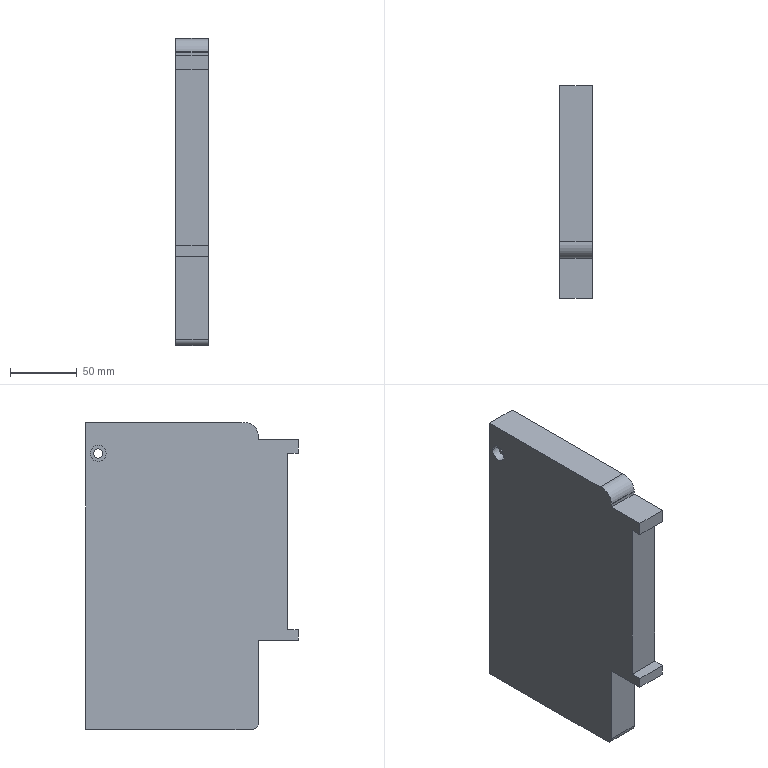Component | SolidWorks | 11-2 | 1 solid | 36 faces | box 24 x 159.37 x 230.25 mm | volume 437688 mm3 | plane 25 | cylinder 11 | commonest cylinder face diameters 20 x3 12 x2 7 x2 24 x2 4 x1 9.34 x1
STEP:
#1=COLOUR_RGB('',0.7922,0.8196,0.9333);
#2=FILL_AREA_STYLE_COLOUR('',#1);
#3=FILL_AREA_STYLE('',(#2));
#4=SURFACE_STYLE_FILL_AREA(#3);
#5=SURFACE_SIDE_STYLE('',(#4));
#6=SURFACE_STYLE_USAGE(.BOTH.,#5);
#7=PRESENTATION_STYLE_ASSIGNMENT((#6));
#8=CARTESIAN_POINT('',(-7.758,16.141,29.439));
#9=VERTEX_POINT('',#8);
#10=CARTESIAN_POINT('',(-7.758,16.614,29.439));
#11=VERTEX_POINT('',#10);
#12=CARTESIAN_POINT('',(-7.758,16.378,29.439));
#13=DIRECTION('',(1.,0.,-0.));
#14=DIRECTION('',(0.,-1.,0.));
#15=AXIS2_PLACEMENT_3D('',#12,#13,#14);
#16=CIRCLE('',#15,0.2362);
#17=EDGE_CURVE('',#9,#11,#16,.T.);
#18=ORIENTED_EDGE('',*,*,#17,.T.);
#19=CARTESIAN_POINT('',(-7.994,16.614,29.439));
#20=VERTEX_POINT('',#19);
#21=CARTESIAN_POINT('',(-7.089,16.614,29.439));
#22=DIRECTION('',(-1.,-0.,0.));
#23=VECTOR('',#22,39.37);
#24=LINE('',#21,#23);
#25=EDGE_CURVE('',#11,#20,#24,.T.);
#26=ORIENTED_EDGE('',*,*,#25,.T.);
#27=CARTESIAN_POINT('',(-7.994,16.141,29.439));
#28=VERTEX_POINT('',#27);
#29=CARTESIAN_POINT('',(-7.994,16.378,29.439));
#30=DIRECTION('',(-1.,-0.,0.));
#31=DIRECTION('',(0.,-1.,0.));
#32=AXIS2_PLACEMENT_3D('',#29,#30,#31);
#33=CIRCLE('',#32,0.2362);
#34=EDGE_CURVE('',#20,#28,#33,.T.);
#35=ORIENTED_EDGE('',*,*,#34,.T.);
#36=CARTESIAN_POINT('',(-7.089,16.141,29.439));
#37=DIRECTION('',(-1.,-0.,0.));
#38=VECTOR('',#37,39.37);
#39=LINE('',#36,#38);
#40=EDGE_CURVE('',#9,#28,#39,.T.);
#41=ORIENTED_EDGE('',*,*,#40,.F.);
#42=EDGE_LOOP('',(#18,#26,#35,#41));
#43=FACE_OUTER_BOUND('',#42,.T.);
#44=CARTESIAN_POINT('',(-7.089,16.378,29.439));
#45=DIRECTION('',(-1.,-0.,0.));
#46=DIRECTION('',(0.,-1.,0.));
#47=AXIS2_PLACEMENT_3D('',#44,#45,#46);
#48=CYLINDRICAL_SURFACE('',#47,0.2362);
#49=ADVANCED_FACE('',(#43),#48,.F.);
#50=CARTESIAN_POINT('',(-7.049,11.653,29.959));
#51=VERTEX_POINT('',#50);
#52=CARTESIAN_POINT('',(-7.049,11.653,29.95));
#53=VERTEX_POINT('',#52);
#54=CARTESIAN_POINT('',(-7.049,12.047,29.959));
#55=DIRECTION('',(1.,0.,-0.));
#56=DIRECTION('',(0.,1.,0.));
#57=AXIS2_PLACEMENT_3D('',#54,#55,#56);
#58=CIRCLE('',#57,0.3937);
#59=EDGE_CURVE('',#51,#53,#58,.T.);
#60=ORIENTED_EDGE('',*,*,#59,.F.);
#61=CARTESIAN_POINT('',(-7.994,11.653,29.959));
#62=VERTEX_POINT('',#61);
#63=CARTESIAN_POINT('',(-7.049,11.653,29.959));
#64=DIRECTION('',(-1.,-0.,0.));
#65=VECTOR('',#64,39.37);
#66=LINE('',#63,#65);
#67=EDGE_CURVE('',#51,#62,#66,.T.);
#68=ORIENTED_EDGE('',*,*,#67,.T.);
#69=CARTESIAN_POINT('',(-7.994,11.653,29.95));
#70=VERTEX_POINT('',#69);
#71=CARTESIAN_POINT('',(-7.994,12.047,29.959));
#72=DIRECTION('',(1.,0.,-0.));
#73=DIRECTION('',(0.,1.,0.));
#74=AXIS2_PLACEMENT_3D('',#71,#72,#73);
#75=CIRCLE('',#74,0.3937);
#76=EDGE_CURVE('',#62,#70,#75,.T.);
#77=ORIENTED_EDGE('',*,*,#76,.T.);
#78=CARTESIAN_POINT('',(-7.049,11.653,29.95));
#79=DIRECTION('',(-1.,-0.,0.));
#80=VECTOR('',#79,39.37);
#81=LINE('',#78,#80);
#82=EDGE_CURVE('',#53,#70,#81,.T.);
#83=ORIENTED_EDGE('',*,*,#82,.F.);
#84=EDGE_LOOP('',(#60,#68,#77,#83));
#85=FACE_OUTER_BOUND('',#84,.T.);
#86=CARTESIAN_POINT('',(-7.049,12.047,29.959));
#87=DIRECTION('',(-1.,-0.,0.));
#88=DIRECTION('',(0.,-1.,0.));
#89=AXIS2_PLACEMENT_3D('',#86,#87,#88);
#90=CYLINDRICAL_SURFACE('',#89,0.3937);
#91=ADVANCED_FACE('',(#85),#90,.T.);
#92=CARTESIAN_POINT('',(-7.758,16.24,29.439));
#93=VERTEX_POINT('',#92);
#94=CARTESIAN_POINT('',(-7.758,16.515,29.439));
#95=VERTEX_POINT('',#94);
#96=CARTESIAN_POINT('',(-7.758,16.378,29.439));
#97=DIRECTION('',(1.,0.,-0.));
#98=DIRECTION('',(0.,-1.,0.));
#99=AXIS2_PLACEMENT_3D('',#96,#97,#98);
#100=CIRCLE('',#99,0.1378);
#101=EDGE_CURVE('',#93,#95,#100,.T.);
#102=ORIENTED_EDGE('',*,*,#101,.F.);
#103=CARTESIAN_POINT('',(-7.049,16.24,29.439));
#104=VERTEX_POINT('',#103);
#105=CARTESIAN_POINT('',(-13.151,16.24,29.439));
#106=DIRECTION('',(1.,0.,-0.));
#107=VECTOR('',#106,39.37);
#108=LINE('',#105,#107);
#109=EDGE_CURVE('',#93,#104,#108,.T.);
#110=ORIENTED_EDGE('',*,*,#109,.T.);
#111=CARTESIAN_POINT('',(-7.049,16.515,29.439));
#112=VERTEX_POINT('',#111);
#113=CARTESIAN_POINT('',(-7.049,16.378,29.439));
#114=DIRECTION('',(1.,0.,-0.));
#115=DIRECTION('',(0.,1.,0.));
#116=AXIS2_PLACEMENT_3D('',#113,#114,#115);
#117=CIRCLE('',#116,0.1378);
#118=EDGE_CURVE('',#104,#112,#117,.T.);
#119=ORIENTED_EDGE('',*,*,#118,.T.);
#120=CARTESIAN_POINT('',(-13.151,16.515,29.439));
#121=DIRECTION('',(1.,0.,-0.));
#122=VECTOR('',#121,39.37);
#123=LINE('',#120,#122);
#124=EDGE_CURVE('',#95,#112,#123,.T.);
#125=ORIENTED_EDGE('',*,*,#124,.F.);
#126=EDGE_LOOP('',(#102,#110,#119,#125));
#127=FACE_OUTER_BOUND('',#126,.T.);
#128=CARTESIAN_POINT('',(-13.151,16.378,29.439));
#129=DIRECTION('',(1.,0.,-0.));
#130=DIRECTION('',(0.,1.,0.));
#131=AXIS2_PLACEMENT_3D('',#128,#129,#130);
#132=CYLINDRICAL_SURFACE('',#131,0.1378);
#133=ADVANCED_FACE('',(#127),#132,.F.);
#134=CARTESIAN_POINT('',(-7.049,15.905,29.439));
#135=VERTEX_POINT('',#134);
#136=CARTESIAN_POINT('',(-7.049,16.31,28.971));
#137=VERTEX_POINT('',#136);
#138=CARTESIAN_POINT('',(-7.049,16.378,29.439));
#139=DIRECTION('',(1.,0.,-0.));
#140=DIRECTION('',(0.,1.,0.));
#141=AXIS2_PLACEMENT_3D('',#138,#139,#140);
#142=CIRCLE('',#141,0.4724);
#143=EDGE_CURVE('',#135,#137,#142,.T.);
#144=ORIENTED_EDGE('',*,*,#143,.F.);
#145=CARTESIAN_POINT('',(-7.6,15.905,29.439));
#146=VERTEX_POINT('',#145);
#147=CARTESIAN_POINT('',(-7.049,15.905,29.439));
#148=DIRECTION('',(-1.,-0.,0.));
#149=VECTOR('',#148,39.37);
#150=LINE('',#147,#149);
#151=EDGE_CURVE('',#135,#146,#150,.T.);
#152=ORIENTED_EDGE('',*,*,#151,.T.);
#153=CARTESIAN_POINT('',(-7.6,16.31,28.971));
#154=VERTEX_POINT('',#153);
#155=CARTESIAN_POINT('',(-7.6,16.378,29.439));
#156=DIRECTION('',(1.,0.,-0.));
#157=DIRECTION('',(0.,-1.,0.));
#158=AXIS2_PLACEMENT_3D('',#155,#156,#157);
#159=CIRCLE('',#158,0.4724);
#160=EDGE_CURVE('',#146,#154,#159,.T.);
#161=ORIENTED_EDGE('',*,*,#160,.T.);
#162=CARTESIAN_POINT('',(-7.049,16.31,28.971));
#163=DIRECTION('',(-1.,-0.,0.));
#164=VECTOR('',#163,39.37);
#165=LINE('',#162,#164);
#166=EDGE_CURVE('',#137,#154,#165,.T.);
#167=ORIENTED_EDGE('',*,*,#166,.F.);
#168=EDGE_LOOP('',(#144,#152,#161,#167));
#169=FACE_OUTER_BOUND('',#168,.T.);
#170=CARTESIAN_POINT('',(-7.049,16.378,29.439));
#171=DIRECTION('',(-1.,-0.,0.));
#172=DIRECTION('',(0.,-1.,0.));
#173=AXIS2_PLACEMENT_3D('',#170,#171,#172);
#174=CYLINDRICAL_SURFACE('',#173,0.4724);
#175=ADVANCED_FACE('',(#169),#174,.T.);
#176=ORIENTED_EDGE('',*,*,#151,.F.);
#177=CARTESIAN_POINT('',(-7.049,16.378,29.911));
#178=VERTEX_POINT('',#177);
#179=CARTESIAN_POINT('',(-7.049,16.378,29.439));
#180=DIRECTION('',(1.,0.,-0.));
#181=DIRECTION('',(0.,1.,0.));
#182=AXIS2_PLACEMENT_3D('',#179,#180,#181);
#183=CIRCLE('',#182,0.4724);
#184=EDGE_CURVE('',#178,#135,#183,.T.);
#185=ORIENTED_EDGE('',*,*,#184,.F.);
#186=CARTESIAN_POINT('',(-7.6,16.378,29.911));
#187=VERTEX_POINT('',#186);
#188=CARTESIAN_POINT('',(-7.049,16.378,29.911));
#189=DIRECTION('',(-1.,-0.,0.));
#190=VECTOR('',#189,39.37);
#191=LINE('',#188,#190);
#192=EDGE_CURVE('',#178,#187,#191,.T.);
#193=ORIENTED_EDGE('',*,*,#192,.T.);
#194=CARTESIAN_POINT('',(-7.6,16.378,29.439));
#195=DIRECTION('',(1.,0.,-0.));
#196=DIRECTION('',(0.,-1.,0.));
#197=AXIS2_PLACEMENT_3D('',#194,#195,#196);
#198=CIRCLE('',#197,0.4724);
#199=EDGE_CURVE('',#187,#146,#198,.T.);
#200=ORIENTED_EDGE('',*,*,#199,.T.);
#201=EDGE_LOOP('',(#176,#185,#193,#200));
#202=FACE_OUTER_BOUND('',#201,.T.);
#203=CARTESIAN_POINT('',(-7.049,16.378,29.439));
#204=DIRECTION('',(-1.,-0.,0.));
#205=DIRECTION('',(0.,-1.,0.));
#206=AXIS2_PLACEMENT_3D('',#203,#204,#205);
#207=CYLINDRICAL_SURFACE('',#206,0.4724);
#208=ADVANCED_FACE('',(#202),#207,.T.);
#209=CARTESIAN_POINT('',(-7.6,16.378,28.893));
#210=VERTEX_POINT('',#209);
#211=CARTESIAN_POINT('',(-7.6,16.299,28.893));
#212=DIRECTION('',(-1.,-0.,0.));
#213=DIRECTION('',(0.,-1.,0.));
#214=AXIS2_PLACEMENT_3D('',#211,#212,#213);
#215=CIRCLE('',#214,0.07874);
#216=EDGE_CURVE('',#154,#210,#215,.T.);
#217=ORIENTED_EDGE('',*,*,#216,.T.);
#218=CARTESIAN_POINT('',(-7.049,16.378,28.893));
#219=VERTEX_POINT('',#218);
#220=CARTESIAN_POINT('',(-7.049,16.378,28.893));
#221=DIRECTION('',(-1.,-0.,0.));
#222=VECTOR('',#221,39.37);
#223=LINE('',#220,#222);
#224=EDGE_CURVE('',#219,#210,#223,.T.);
#225=ORIENTED_EDGE('',*,*,#224,.F.);
#226=CARTESIAN_POINT('',(-7.049,16.299,28.893));
#227=DIRECTION('',(-1.,-0.,0.));
#228=DIRECTION('',(0.,1.,0.));
#229=AXIS2_PLACEMENT_3D('',#226,#227,#228);
#230=CIRCLE('',#229,0.07874);
#231=EDGE_CURVE('',#137,#219,#230,.T.);
#232=ORIENTED_EDGE('',*,*,#231,.F.);
#233=ORIENTED_EDGE('',*,*,#166,.T.);
#234=EDGE_LOOP('',(#217,#225,#232,#233));
#235=FACE_OUTER_BOUND('',#234,.T.);
#236=CARTESIAN_POINT('',(-7.049,16.299,28.893));
#237=DIRECTION('',(-1.,-0.,0.));
#238=DIRECTION('',(0.,-1.,0.));
#239=AXIS2_PLACEMENT_3D('',#236,#237,#238);
#240=CYLINDRICAL_SURFACE('',#239,0.07874);
#241=ADVANCED_FACE('',(#235),#240,.F.);
#242=ORIENTED_EDGE('',*,*,#224,.T.);
#243=CARTESIAN_POINT('',(-7.6,16.378,21.603));
#244=VERTEX_POINT('',#243);
#245=CARTESIAN_POINT('',(-7.6,16.378,21.603));
#246=DIRECTION('',(-0.,-0.,-1.));
#247=VECTOR('',#246,39.37);
#248=LINE('',#245,#247);
#249=EDGE_CURVE('',#210,#244,#248,.T.);
#250=ORIENTED_EDGE('',*,*,#249,.T.);
#251=CARTESIAN_POINT('',(-7.049,16.378,21.603));
#252=VERTEX_POINT('',#251);
#253=CARTESIAN_POINT('',(-7.049,16.378,21.603));
#254=DIRECTION('',(-1.,-0.,0.));
#255=VECTOR('',#254,39.37);
#256=LINE('',#253,#255);
#257=EDGE_CURVE('',#252,#244,#256,.T.);
#258=ORIENTED_EDGE('',*,*,#257,.F.);
#259=CARTESIAN_POINT('',(-7.049,16.378,26.958));
#260=DIRECTION('',(0.,0.,1.));
#261=VECTOR('',#260,39.37);
#262=LINE('',#259,#261);
#263=EDGE_CURVE('',#252,#219,#262,.T.);
#264=ORIENTED_EDGE('',*,*,#263,.T.);
#265=EDGE_LOOP('',(#242,#250,#258,#264));
#266=FACE_OUTER_BOUND('',#265,.T.);
#267=CARTESIAN_POINT('',(-7.049,16.378,26.958));
#268=DIRECTION('',(0.,-1.,0.));
#269=DIRECTION('',(1.,0.,-0.));
#270=AXIS2_PLACEMENT_3D('',#267,#268,#269);
#271=PLANE('',#270);
#272=ADVANCED_FACE('',(#266),#271,.T.);
#273=CARTESIAN_POINT('',(-7.6,12.637,21.603));
#274=VERTEX_POINT('',#273);
#275=CARTESIAN_POINT('',(-7.6,16.378,21.603));
#276=DIRECTION('',(0.,-1.,0.));
#277=VECTOR('',#276,39.37);
#278=LINE('',#275,#277);
#279=EDGE_CURVE('',#244,#274,#278,.T.);
#280=ORIENTED_EDGE('',*,*,#279,.T.);
#281=CARTESIAN_POINT('',(-7.049,12.637,21.603));
#282=VERTEX_POINT('',#281);
#283=CARTESIAN_POINT('',(-7.049,12.637,21.603));
#284=DIRECTION('',(-1.,-0.,0.));
#285=VECTOR('',#284,39.37);
#286=LINE('',#283,#285);
#287=EDGE_CURVE('',#282,#274,#286,.T.);
#288=ORIENTED_EDGE('',*,*,#287,.F.);
#289=CARTESIAN_POINT('',(-7.049,14.527,21.603));
#290=DIRECTION('',(0.,-1.,0.));
#291=VECTOR('',#290,39.37);
#292=LINE('',#289,#291);
#293=EDGE_CURVE('',#252,#282,#292,.T.);
#294=ORIENTED_EDGE('',*,*,#293,.F.);
#295=ORIENTED_EDGE('',*,*,#257,.T.);
#296=EDGE_LOOP('',(#280,#288,#294,#295));
#297=FACE_OUTER_BOUND('',#296,.T.);
#298=CARTESIAN_POINT('',(-7.049,14.527,21.603));
#299=DIRECTION('',(-0.,-0.,-1.));
#300=DIRECTION('',(-0.,1.,-0.));
#301=AXIS2_PLACEMENT_3D('',#298,#299,#300);
#302=PLANE('',#301);
#303=ADVANCED_FACE('',(#297),#302,.F.);
#304=ORIENTED_EDGE('',*,*,#287,.T.);
#305=CARTESIAN_POINT('',(-7.6,12.637,23.847));
#306=VERTEX_POINT('',#305);
#307=CARTESIAN_POINT('',(-7.6,12.637,23.847));
#308=DIRECTION('',(0.,0.,1.));
#309=VECTOR('',#308,39.37);
#310=LINE('',#307,#309);
#311=EDGE_CURVE('',#274,#306,#310,.T.);
#312=ORIENTED_EDGE('',*,*,#311,.T.);
#313=CARTESIAN_POINT('',(-7.049,12.637,23.847));
#314=VERTEX_POINT('',#313);
#315=CARTESIAN_POINT('',(-7.049,12.637,23.847));
#316=DIRECTION('',(-1.,-0.,0.));
#317=VECTOR('',#316,39.37);
#318=LINE('',#315,#317);
#319=EDGE_CURVE('',#314,#306,#318,.T.);
#320=ORIENTED_EDGE('',*,*,#319,.F.);
#321=CARTESIAN_POINT('',(-7.049,12.637,26.958));
#322=DIRECTION('',(-0.,-0.,-1.));
#323=VECTOR('',#322,39.37);
#324=LINE('',#321,#323);
#325=EDGE_CURVE('',#314,#282,#324,.T.);
#326=ORIENTED_EDGE('',*,*,#325,.T.);
#327=EDGE_LOOP('',(#304,#312,#320,#326));
#328=FACE_OUTER_BOUND('',#327,.T.);
#329=CARTESIAN_POINT('',(-7.049,12.637,26.958));
#330=DIRECTION('',(-0.,1.,-0.));
#331=DIRECTION('',(0.,0.,1.));
#332=AXIS2_PLACEMENT_3D('',#329,#330,#331);
#333=PLANE('',#332);
#334=ADVANCED_FACE('',(#328),#333,.T.);
#335=CARTESIAN_POINT('',(-7.6,12.244,24.241));
#336=VERTEX_POINT('',#335);
#337=CARTESIAN_POINT('',(-7.6,12.244,23.847));
#338=DIRECTION('',(1.,0.,-0.));
#339=DIRECTION('',(0.,-1.,0.));
#340=AXIS2_PLACEMENT_3D('',#337,#338,#339);
#341=CIRCLE('',#340,0.3937);
#342=EDGE_CURVE('',#306,#336,#341,.T.);
#343=ORIENTED_EDGE('',*,*,#342,.T.);
#344=CARTESIAN_POINT('',(-7.049,12.244,24.241));
#345=VERTEX_POINT('',#344);
#346=CARTESIAN_POINT('',(-7.049,12.244,24.241));
#347=DIRECTION('',(-1.,-0.,0.));
#348=VECTOR('',#347,39.37);
#349=LINE('',#346,#348);
#350=EDGE_CURVE('',#345,#336,#349,.T.);
#351=ORIENTED_EDGE('',*,*,#350,.F.);
#352=CARTESIAN_POINT('',(-7.049,12.244,23.847));
#353=DIRECTION('',(1.,0.,-0.));
#354=DIRECTION('',(0.,1.,0.));
#355=AXIS2_PLACEMENT_3D('',#352,#353,#354);
#356=CIRCLE('',#355,0.3937);
#357=EDGE_CURVE('',#314,#345,#356,.T.);
#358=ORIENTED_EDGE('',*,*,#357,.F.);
#359=ORIENTED_EDGE('',*,*,#319,.T.);
#360=EDGE_LOOP('',(#343,#351,#358,#359));
#361=FACE_OUTER_BOUND('',#360,.T.);
#362=CARTESIAN_POINT('',(-7.049,12.244,23.847));
#363=DIRECTION('',(-1.,-0.,0.));
#364=DIRECTION('',(0.,-1.,0.));
#365=AXIS2_PLACEMENT_3D('',#362,#363,#364);
#366=CYLINDRICAL_SURFACE('',#365,0.3937);
#367=ADVANCED_FACE('',(#361),#366,.T.);
#368=CARTESIAN_POINT('',(-7.6,11.102,24.241));
#369=VERTEX_POINT('',#368);
#370=CARTESIAN_POINT('',(-7.6,12.244,24.241));
#371=DIRECTION('',(0.,-1.,0.));
#372=VECTOR('',#371,39.37);
#373=LINE('',#370,#372);
#374=EDGE_CURVE('',#336,#369,#373,.T.);
#375=ORIENTED_EDGE('',*,*,#374,.T.);
#376=CARTESIAN_POINT('',(-7.049,11.102,24.241));
#377=VERTEX_POINT('',#376);
#378=CARTESIAN_POINT('',(-7.049,11.102,24.241));
#379=DIRECTION('',(-1.,-0.,0.));
#380=VECTOR('',#379,39.37);
#381=LINE('',#378,#380);
#382=EDGE_CURVE('',#377,#369,#381,.T.);
#383=ORIENTED_EDGE('',*,*,#382,.F.);
#384=CARTESIAN_POINT('',(-7.049,14.527,24.241));
#385=DIRECTION('',(0.,-1.,0.));
#386=VECTOR('',#385,39.37);
#387=LINE('',#384,#386);
#388=EDGE_CURVE('',#345,#377,#387,.T.);
#389=ORIENTED_EDGE('',*,*,#388,.F.);
#390=ORIENTED_EDGE('',*,*,#350,.T.);
#391=EDGE_LOOP('',(#375,#383,#389,#390));
#392=FACE_OUTER_BOUND('',#391,.T.);
#393=CARTESIAN_POINT('',(-7.049,14.527,24.241));
#394=DIRECTION('',(-0.,-0.,-1.));
#395=DIRECTION('',(-1.,-0.,0.));
#396=AXIS2_PLACEMENT_3D('',#393,#394,#395);
#397=PLANE('',#396);
#398=ADVANCED_FACE('',(#392),#397,.F.);
#399=ORIENTED_EDGE('',*,*,#382,.T.);
#400=CARTESIAN_POINT('',(-7.6,11.102,29.445));
#401=VERTEX_POINT('',#400);
#402=CARTESIAN_POINT('',(-7.6,11.102,29.445));
#403=DIRECTION('',(0.,0.,1.));
#404=VECTOR('',#403,39.37);
#405=LINE('',#402,#404);
#406=EDGE_CURVE('',#369,#401,#405,.T.);
#407=ORIENTED_EDGE('',*,*,#406,.T.);
#408=CARTESIAN_POINT('',(-7.049,11.102,29.445));
#409=VERTEX_POINT('',#408);
#410=CARTESIAN_POINT('',(-7.049,11.102,29.445));
#411=DIRECTION('',(-1.,-0.,0.));
#412=VECTOR('',#411,39.37);
#413=LINE('',#410,#412);
#414=EDGE_CURVE('',#409,#401,#413,.T.);
#415=ORIENTED_EDGE('',*,*,#414,.F.);
#416=CARTESIAN_POINT('',(-7.049,11.102,26.958));
#417=DIRECTION('',(-0.,-0.,-1.));
#418=VECTOR('',#417,39.37);
#419=LINE('',#416,#418);
#420=EDGE_CURVE('',#409,#377,#419,.T.);
#421=ORIENTED_EDGE('',*,*,#420,.T.);
#422=EDGE_LOOP('',(#399,#407,#415,#421));
#423=FACE_OUTER_BOUND('',#422,.T.);
#424=CARTESIAN_POINT('',(-7.049,11.102,26.958));
#425=DIRECTION('',(-0.,1.,-0.));
#426=DIRECTION('',(-1.,-0.,0.));
#427=AXIS2_PLACEMENT_3D('',#424,#425,#426);
#428=PLANE('',#427);
#429=ADVANCED_FACE('',(#423),#428,.T.);
#430=ORIENTED_EDGE('',*,*,#414,.T.);
#431=CARTESIAN_POINT('',(-7.6,11.968,29.445));
#432=VERTEX_POINT('',#431);
#433=CARTESIAN_POINT('',(-7.6,11.968,29.445));
#434=DIRECTION('',(-0.,1.,-0.));
#435=VECTOR('',#434,39.37);
#436=LINE('',#433,#435);
#437=EDGE_CURVE('',#401,#432,#436,.T.);
#438=ORIENTED_EDGE('',*,*,#437,.T.);
#439=CARTESIAN_POINT('',(-7.049,11.968,29.445));
#440=VERTEX_POINT('',#439);
#441=CARTESIAN_POINT('',(-7.049,11.968,29.445));
#442=DIRECTION('',(-1.,-0.,0.));
#443=VECTOR('',#442,39.37);
#444=LINE('',#441,#443);
#445=EDGE_CURVE('',#440,#432,#444,.T.);
#446=ORIENTED_EDGE('',*,*,#445,.F.);
#447=CARTESIAN_POINT('',(-7.049,14.527,29.445));
#448=DIRECTION('',(0.,-1.,0.));
#449=VECTOR('',#448,39.37);
#450=LINE('',#447,#449);
#451=EDGE_CURVE('',#440,#409,#450,.T.);
#452=ORIENTED_EDGE('',*,*,#451,.T.);
#453=EDGE_LOOP('',(#430,#438,#446,#452));
#454=FACE_OUTER_BOUND('',#453,.T.);
#455=CARTESIAN_POINT('',(-7.049,14.527,29.445));
#456=DIRECTION('',(-0.,-0.,-1.));
#457=DIRECTION('',(-1.,-0.,0.));
#458=AXIS2_PLACEMENT_3D('',#455,#456,#457);
#459=PLANE('',#458);
#460=ADVANCED_FACE('',(#454),#459,.T.);
#461=ORIENTED_EDGE('',*,*,#445,.T.);
#462=CARTESIAN_POINT('',(-7.6,11.968,30.028));
#463=VERTEX_POINT('',#462);
#464=CARTESIAN_POINT('',(-7.6,11.968,30.028));
#465=DIRECTION('',(0.,0.,1.));
#466=VECTOR('',#465,39.37);
#467=LINE('',#464,#466);
#468=EDGE_CURVE('',#432,#463,#467,.T.);
#469=ORIENTED_EDGE('',*,*,#468,.T.);
#470=CARTESIAN_POINT('',(-7.049,11.968,30.028));
#471=VERTEX_POINT('',#470);
#472=CARTESIAN_POINT('',(-7.049,11.968,30.028));
#473=DIRECTION('',(-1.,-0.,0.));
#474=VECTOR('',#473,39.37);
#475=LINE('',#472,#474);
#476=EDGE_CURVE('',#471,#463,#475,.T.);
#477=ORIENTED_EDGE('',*,*,#476,.F.);
#478=CARTESIAN_POINT('',(-7.049,11.968,26.958));
#479=DIRECTION('',(-0.,-0.,-1.));
#480=VECTOR('',#479,39.37);
#481=LINE('',#478,#480);
#482=EDGE_CURVE('',#471,#440,#481,.T.);
#483=ORIENTED_EDGE('',*,*,#482,.T.);
#484=EDGE_LOOP('',(#461,#469,#477,#483));
#485=FACE_OUTER_BOUND('',#484,.T.);
#486=CARTESIAN_POINT('',(-7.049,11.968,26.958));
#487=DIRECTION('',(-0.,1.,-0.));
#488=DIRECTION('',(-1.,-0.,0.));
#489=AXIS2_PLACEMENT_3D('',#486,#487,#488);
#490=PLANE('',#489);
#491=ADVANCED_FACE('',(#485),#490,.T.);
#492=CARTESIAN_POINT('',(-7.6,16.378,30.028));
#493=VERTEX_POINT('',#492);
#494=CARTESIAN_POINT('',(-7.6,11.968,30.028));
#495=DIRECTION('',(-0.,1.,-0.));
#496=VECTOR('',#495,39.37);
#497=LINE('',#494,#496);
#498=EDGE_CURVE('',#463,#493,#497,.T.);
#499=ORIENTED_EDGE('',*,*,#498,.T.);
#500=CARTESIAN_POINT('',(-7.049,16.378,30.028));
#501=VERTEX_POINT('',#500);
#502=CARTESIAN_POINT('',(-7.049,16.378,30.028));
#503=DIRECTION('',(-1.,-0.,0.));
#504=VECTOR('',#503,39.37);
#505=LINE('',#502,#504);
#506=EDGE_CURVE('',#501,#493,#505,.T.);
#507=ORIENTED_EDGE('',*,*,#506,.F.);
#508=CARTESIAN_POINT('',(-7.049,14.527,30.028));
#509=DIRECTION('',(-0.,1.,-0.));
#510=VECTOR('',#509,39.37);
#511=LINE('',#508,#510);
#512=EDGE_CURVE('',#471,#501,#511,.T.);
#513=ORIENTED_EDGE('',*,*,#512,.F.);
#514=ORIENTED_EDGE('',*,*,#476,.T.);
#515=EDGE_LOOP('',(#499,#507,#513,#514));
#516=FACE_OUTER_BOUND('',#515,.T.);
#517=CARTESIAN_POINT('',(-7.049,14.527,30.028));
#518=DIRECTION('',(0.,0.,1.));
#519=DIRECTION('',(0.,-1.,0.));
#520=AXIS2_PLACEMENT_3D('',#517,#518,#519);
#521=PLANE('',#520);
#522=ADVANCED_FACE('',(#516),#521,.F.);
#523=ORIENTED_EDGE('',*,*,#506,.T.);
#524=CARTESIAN_POINT('',(-7.6,16.378,29.911));
#525=DIRECTION('',(-0.,-0.,-1.));
#526=VECTOR('',#525,39.37);
#527=LINE('',#524,#526);
#528=EDGE_CURVE('',#493,#187,#527,.T.);
#529=ORIENTED_EDGE('',*,*,#528,.T.);
#530=ORIENTED_EDGE('',*,*,#192,.F.);
#531=CARTESIAN_POINT('',(-7.049,16.378,26.958));
#532=DIRECTION('',(0.,0.,1.));
#533=VECTOR('',#532,39.37);
#534=LINE('',#531,#533);
#535=EDGE_CURVE('',#178,#501,#534,.T.);
#536=ORIENTED_EDGE('',*,*,#535,.T.);
#537=EDGE_LOOP('',(#523,#529,#530,#536));
#538=FACE_OUTER_BOUND('',#537,.T.);
#539=CARTESIAN_POINT('',(-7.049,16.378,26.958));
#540=DIRECTION('',(0.,-1.,0.));
#541=DIRECTION('',(-0.,-0.,-1.));
#542=AXIS2_PLACEMENT_3D('',#539,#540,#541);
#543=PLANE('',#542);
#544=ADVANCED_FACE('',(#538),#543,.T.);
#545=ORIENTED_EDGE('',*,*,#109,.F.);
#546=CARTESIAN_POINT('',(-7.758,16.378,29.439));
#547=DIRECTION('',(1.,0.,-0.));
#548=DIRECTION('',(0.,-1.,0.));
#549=AXIS2_PLACEMENT_3D('',#546,#547,#548);
#550=CIRCLE('',#549,0.1378);
#551=EDGE_CURVE('',#95,#93,#550,.T.);
#552=ORIENTED_EDGE('',*,*,#551,.F.);
#553=ORIENTED_EDGE('',*,*,#124,.T.);
#554=CARTESIAN_POINT('',(-7.049,16.378,29.439));
#555=DIRECTION('',(1.,0.,-0.));
#556=DIRECTION('',(0.,1.,0.));
#557=AXIS2_PLACEMENT_3D('',#554,#555,#556);
#558=CIRCLE('',#557,0.1378);
#559=EDGE_CURVE('',#112,#104,#558,.T.);
#560=ORIENTED_EDGE('',*,*,#559,.T.);
#561=EDGE_LOOP('',(#545,#552,#553,#560));
#562=FACE_OUTER_BOUND('',#561,.T.);
#563=CARTESIAN_POINT('',(-13.151,16.378,29.439));
#564=DIRECTION('',(1.,0.,-0.));
#565=DIRECTION('',(0.,1.,0.));
#566=AXIS2_PLACEMENT_3D('',#563,#564,#565);
#567=CYLINDRICAL_SURFACE('',#566,0.1378);
#568=ADVANCED_FACE('',(#562),#567,.F.);
#569=CARTESIAN_POINT('',(-7.994,12.134,30.343));
#570=VERTEX_POINT('',#569);
#571=CARTESIAN_POINT('',(-7.994,16.746,30.343));
#572=VERTEX_POINT('',#571);
#573=CARTESIAN_POINT('',(-7.994,14.527,30.343));
#574=DIRECTION('',(-0.,1.,-0.));
#575=VECTOR('',#574,39.37);
#576=LINE('',#573,#575);
#577=EDGE_CURVE('',#570,#572,#576,.T.);
#578=ORIENTED_EDGE('',*,*,#577,.F.);
#579=CARTESIAN_POINT('',(-7.049,12.134,30.343));
#580=VERTEX_POINT('',#579);
#581=CARTESIAN_POINT('',(-7.049,12.134,30.343));
#582=DIRECTION('',(-1.,-0.,0.));
#583=VECTOR('',#582,39.37);
#584=LINE('',#581,#583);
#585=EDGE_CURVE('',#580,#570,#584,.T.);
#586=ORIENTED_EDGE('',*,*,#585,.F.);
#587=CARTESIAN_POINT('',(-7.049,16.746,30.343));
#588=VERTEX_POINT('',#587);
#589=CARTESIAN_POINT('',(-7.049,14.527,30.343));
#590=DIRECTION('',(-0.,1.,-0.));
#591=VECTOR('',#590,39.37);
#592=LINE('',#589,#591);
#593=EDGE_CURVE('',#580,#588,#592,.T.);
#594=ORIENTED_EDGE('',*,*,#593,.T.);
#595=CARTESIAN_POINT('',(-7.049,16.746,30.343));
#596=DIRECTION('',(-1.,-0.,0.));
#597=VECTOR('',#596,39.37);
#598=LINE('',#595,#597);
#599=EDGE_CURVE('',#588,#572,#598,.T.);
#600=ORIENTED_EDGE('',*,*,#599,.T.);
#601=EDGE_LOOP('',(#578,#586,#594,#600));
#602=FACE_OUTER_BOUND('',#601,.T.);
#603=CARTESIAN_POINT('',(-7.049,14.527,30.343));
#604=DIRECTION('',(0.,0.,1.));
#605=DIRECTION('',(0.,-1.,0.));
#606=AXIS2_PLACEMENT_3D('',#603,#604,#605);
#607=PLANE('',#606);
#608=ADVANCED_FACE('',(#602),#607,.T.);
#609=ORIENTED_EDGE('',*,*,#67,.F.);
#610=CARTESIAN_POINT('',(-7.049,12.047,29.959));
#611=DIRECTION('',(1.,0.,-0.));
#612=DIRECTION('',(0.,1.,0.));
#613=AXIS2_PLACEMENT_3D('',#610,#611,#612);
#614=CIRCLE('',#613,0.3937);
#615=EDGE_CURVE('',#580,#51,#614,.T.);
#616=ORIENTED_EDGE('',*,*,#615,.F.);
#617=ORIENTED_EDGE('',*,*,#585,.T.);
#618=CARTESIAN_POINT('',(-7.994,12.047,29.959));
#619=DIRECTION('',(1.,0.,-0.));
#620=DIRECTION('',(0.,1.,0.));
#621=AXIS2_PLACEMENT_3D('',#618,#619,#620);
#622=CIRCLE('',#621,0.3937);
#623=EDGE_CURVE('',#570,#62,#622,.T.);
#624=ORIENTED_EDGE('',*,*,#623,.T.);
#625=EDGE_LOOP('',(#609,#616,#617,#624));
#626=FACE_OUTER_BOUND('',#625,.T.);
#627=CARTESIAN_POINT('',(-7.049,12.047,29.959));
#628=DIRECTION('',(-1.,-0.,0.));
#629=DIRECTION('',(0.,-1.,0.));
#630=AXIS2_PLACEMENT_3D('',#627,#628,#629);
#631=CYLINDRICAL_SURFACE('',#630,0.3937);
#632=ADVANCED_FACE('',(#626),#631,.T.);
#633=CARTESIAN_POINT('',(-7.994,11.653,29.85));
#634=VERTEX_POINT('',#633);
#635=CARTESIAN_POINT('',(-7.994,11.653,26.958));
#636=DIRECTION('',(-0.,-0.,-1.));
#637=VECTOR('',#636,39.37);
#638=LINE('',#635,#637);
#639=EDGE_CURVE('',#70,#634,#638,.T.);
#640=ORIENTED_EDGE('',*,*,#639,.T.);
#641=CARTESIAN_POINT('',(-7.049,11.653,29.85));
#642=VERTEX_POINT('',#641);
#643=CARTESIAN_POINT('',(-7.049,11.653,29.85));
#644=DIRECTION('',(-1.,-0.,0.));
#645=VECTOR('',#644,39.37);
#646=LINE('',#643,#645);
#647=EDGE_CURVE('',#642,#634,#646,.T.);
#648=ORIENTED_EDGE('',*,*,#647,.F.);
#649=CARTESIAN_POINT('',(-7.049,11.653,26.958));
#650=DIRECTION('',(-0.,-0.,-1.));
#651=VECTOR('',#650,39.37);
#652=LINE('',#649,#651);
#653=EDGE_CURVE('',#53,#642,#652,.T.);
#654=ORIENTED_EDGE('',*,*,#653,.F.);
#655=ORIENTED_EDGE('',*,*,#82,.T.);
#656=EDGE_LOOP('',(#640,#648,#654,#655));
#657=FACE_OUTER_BOUND('',#656,.T.);
#658=CARTESIAN_POINT('',(-7.049,11.653,26.958));
#659=DIRECTION('',(-0.,1.,-0.));
#660=DIRECTION('',(-1.,-0.,0.));
#661=AXIS2_PLACEMENT_3D('',#658,#659,#660);
#662=PLANE('',#661);
#663=ADVANCED_FACE('',(#657),#662,.F.);
#664=CARTESIAN_POINT('',(-7.994,10.472,29.85));
#665=VERTEX_POINT('',#664);
#666=CARTESIAN_POINT('',(-7.994,14.527,29.85));
#667=DIRECTION('',(0.,-1.,0.));
#668=VECTOR('',#667,39.37);
#669=LINE('',#666,#668);
#670=EDGE_CURVE('',#634,#665,#669,.T.);
#671=ORIENTED_EDGE('',*,*,#670,.T.);
#672=CARTESIAN_POINT('',(-7.049,10.472,29.85));
#673=VERTEX_POINT('',#672);
#674=CARTESIAN_POINT('',(-7.049,10.472,29.85));
#675=DIRECTION('',(-1.,-0.,0.));
#676=VECTOR('',#675,39.37);
#677=LINE('',#674,#676);
#678=EDGE_CURVE('',#673,#665,#677,.T.);
#679=ORIENTED_EDGE('',*,*,#678,.F.);
#680=CARTESIAN_POINT('',(-7.049,14.527,29.85));
#681=DIRECTION('',(0.,-1.,0.));
#682=VECTOR('',#681,39.37);
#683=LINE('',#680,#682);
#684=EDGE_CURVE('',#642,#673,#683,.T.);
#685=ORIENTED_EDGE('',*,*,#684,.F.);
#686=ORIENTED_EDGE('',*,*,#647,.T.);
#687=EDGE_LOOP('',(#671,#679,#685,#686));
#688=FACE_OUTER_BOUND('',#687,.T.);
#689=CARTESIAN_POINT('',(-7.049,14.527,29.85));
#690=DIRECTION('',(-0.,-0.,-1.));
#691=DIRECTION('',(-1.,-0.,0.));
#692=AXIS2_PLACEMENT_3D('',#689,#690,#691);
#693=PLANE('',#692);
#694=ADVANCED_FACE('',(#688),#693,.F.);
#695=CARTESIAN_POINT('',(-7.994,10.472,29.445));
#696=VERTEX_POINT('',#695);
#697=CARTESIAN_POINT('',(-7.994,10.472,26.958));
#698=DIRECTION('',(0.,0.,1.));
#699=VECTOR('',#698,39.37);
#700=LINE('',#697,#699);
#701=EDGE_CURVE('',#696,#665,#700,.T.);
#702=ORIENTED_EDGE('',*,*,#701,.F.);
#703=CARTESIAN_POINT('',(-7.049,10.472,29.445));
#704=VERTEX_POINT('',#703);
#705=CARTESIAN_POINT('',(-7.049,10.472,29.445));
#706=DIRECTION('',(-1.,-0.,0.));
#707=VECTOR('',#706,39.37);
#708=LINE('',#705,#707);
#709=EDGE_CURVE('',#704,#696,#708,.T.);
#710=ORIENTED_EDGE('',*,*,#709,.F.);
#711=CARTESIAN_POINT('',(-7.049,10.472,26.958));
#712=DIRECTION('',(0.,0.,1.));
#713=VECTOR('',#712,39.37);
#714=LINE('',#711,#713);
#715=EDGE_CURVE('',#704,#673,#714,.T.);
#716=ORIENTED_EDGE('',*,*,#715,.T.);
#717=ORIENTED_EDGE('',*,*,#678,.T.);
#718=EDGE_LOOP('',(#702,#710,#716,#717));
#719=FACE_OUTER_BOUND('',#718,.T.);
#720=CARTESIAN_POINT('',(-7.049,10.472,26.958));
#721=DIRECTION('',(0.,-1.,0.));
#722=DIRECTION('',(1.,0.,-0.));
#723=AXIS2_PLACEMENT_3D('',#720,#721,#722);
#724=PLANE('',#723);
#725=ADVANCED_FACE('',(#719),#724,.T.);
#726=CARTESIAN_POINT('',(-7.994,10.787,29.445));
#727=VERTEX_POINT('',#726);
#728=CARTESIAN_POINT('',(-7.994,14.527,29.445));
#729=DIRECTION('',(0.,-1.,0.));
#730=VECTOR('',#729,39.37);
#731=LINE('',#728,#730);
#732=EDGE_CURVE('',#727,#696,#731,.T.);
#733=ORIENTED_EDGE('',*,*,#732,.F.);
#734=CARTESIAN_POINT('',(-7.049,10.787,29.445));
#735=VERTEX_POINT('',#734);
#736=CARTESIAN_POINT('',(-7.049,10.787,29.445));
#737=DIRECTION('',(-1.,-0.,0.));
#738=VECTOR('',#737,39.37);
#739=LINE('',#736,#738);
#740=EDGE_CURVE('',#735,#727,#739,.T.);
#741=ORIENTED_EDGE('',*,*,#740,.F.);
#742=CARTESIAN_POINT('',(-7.049,14.527,29.445));
#743=DIRECTION('',(0.,-1.,0.));
#744=VECTOR('',#743,39.37);
#745=LINE('',#742,#744);
#746=EDGE_CURVE('',#735,#704,#745,.T.);
#747=ORIENTED_EDGE('',*,*,#746,.T.);
#748=ORIENTED_EDGE('',*,*,#709,.T.);
#749=EDGE_LOOP('',(#733,#741,#747,#748));
#750=FACE_OUTER_BOUND('',#749,.T.);
#751=CARTESIAN_POINT('',(-7.049,14.527,29.445));
#752=DIRECTION('',(-0.,-0.,-1.));
#753=DIRECTION('',(-1.,-0.,0.));
#754=AXIS2_PLACEMENT_3D('',#751,#752,#753);
#755=PLANE('',#754);
#756=ADVANCED_FACE('',(#750),#755,.T.);
#757=CARTESIAN_POINT('',(-7.994,10.787,24.241));
#758=VERTEX_POINT('',#757);
#759=CARTESIAN_POINT('',(-7.994,10.787,26.958));
#760=DIRECTION('',(-0.,-0.,-1.));
#761=VECTOR('',#760,39.37);
#762=LINE('',#759,#761);
#763=EDGE_CURVE('',#727,#758,#762,.T.);
#764=ORIENTED_EDGE('',*,*,#763,.T.);
#765=CARTESIAN_POINT('',(-7.049,10.787,24.241));
#766=VERTEX_POINT('',#765);
#767=CARTESIAN_POINT('',(-7.049,10.787,24.241));
#768=DIRECTION('',(-1.,-0.,0.));
#769=VECTOR('',#768,39.37);
#770=LINE('',#767,#769);
#771=EDGE_CURVE('',#766,#758,#770,.T.);
#772=ORIENTED_EDGE('',*,*,#771,.F.);
#773=CARTESIAN_POINT('',(-7.049,10.787,26.958));
#774=DIRECTION('',(-0.,-0.,-1.));
#775=VECTOR('',#774,39.37);
#776=LINE('',#773,#775);
#777=EDGE_CURVE('',#735,#766,#776,.T.);
#778=ORIENTED_EDGE('',*,*,#777,.F.);
#779=ORIENTED_EDGE('',*,*,#740,.T.);
#780=EDGE_LOOP('',(#764,#772,#778,#779));
#781=FACE_OUTER_BOUND('',#780,.T.);
#782=CARTESIAN_POINT('',(-7.049,10.787,26.958));
#783=DIRECTION('',(-0.,1.,-0.));
#784=DIRECTION('',(-1.,-0.,0.));
#785=AXIS2_PLACEMENT_3D('',#782,#783,#784);
#786=PLANE('',#785);
#787=ADVANCED_FACE('',(#781),#786,.F.);
#788=CARTESIAN_POINT('',(-7.994,10.472,24.241));
#789=VERTEX_POINT('',#788);
#790=CARTESIAN_POINT('',(-7.994,14.527,24.241));
#791=DIRECTION('',(0.,-1.,0.));
#792=VECTOR('',#791,39.37);
#793=LINE('',#790,#792);
#794=EDGE_CURVE('',#758,#789,#793,.T.);
#795=ORIENTED_EDGE('',*,*,#794,.T.);
#796=CARTESIAN_POINT('',(-7.049,10.472,24.241));
#797=VERTEX_POINT('',#796);
#798=CARTESIAN_POINT('',(-7.049,10.472,24.241));
#799=DIRECTION('',(-1.,-0.,0.));
#800=VECTOR('',#799,39.37);
#801=LINE('',#798,#800);
#802=EDGE_CURVE('',#797,#789,#801,.T.);
#803=ORIENTED_EDGE('',*,*,#802,.F.);
#804=CARTESIAN_POINT('',(-7.049,14.527,24.241));
#805=DIRECTION('',(0.,-1.,0.));
#806=VECTOR('',#805,39.37);
#807=LINE('',#804,#806);
#808=EDGE_CURVE('',#766,#797,#807,.T.);
#809=ORIENTED_EDGE('',*,*,#808,.F.);
#810=ORIENTED_EDGE('',*,*,#771,.T.);
#811=EDGE_LOOP('',(#795,#803,#809,#810));
#812=FACE_OUTER_BOUND('',#811,.T.);
#813=CARTESIAN_POINT('',(-7.049,14.527,24.241));
#814=DIRECTION('',(-0.,-0.,-1.));
#815=DIRECTION('',(-1.,-0.,0.));
#816=AXIS2_PLACEMENT_3D('',#813,#814,#815);
#817=PLANE('',#816);
#818=ADVANCED_FACE('',(#812),#817,.F.);
#819=CARTESIAN_POINT('',(-7.994,10.472,23.926));
#820=VERTEX_POINT('',#819);
#821=CARTESIAN_POINT('',(-7.994,10.472,26.958));
#822=DIRECTION('',(0.,0.,1.));
#823=VECTOR('',#822,39.37);
#824=LINE('',#821,#823);
#825=EDGE_CURVE('',#820,#789,#824,.T.);
#826=ORIENTED_EDGE('',*,*,#825,.F.);
#827=CARTESIAN_POINT('',(-7.049,10.472,23.926));
#828=VERTEX_POINT('',#827);
#829=CARTESIAN_POINT('',(-7.049,10.472,23.926));
#830=DIRECTION('',(-1.,-0.,0.));
#831=VECTOR('',#830,39.37);
#832=LINE('',#829,#831);
#833=EDGE_CURVE('',#828,#820,#832,.T.);
#834=ORIENTED_EDGE('',*,*,#833,.F.);
#835=CARTESIAN_POINT('',(-7.049,10.472,26.958));
#836=DIRECTION('',(0.,0.,1.));
#837=VECTOR('',#836,39.37);
#838=LINE('',#835,#837);
#839=EDGE_CURVE('',#828,#797,#838,.T.);
#840=ORIENTED_EDGE('',*,*,#839,.T.);
#841=ORIENTED_EDGE('',*,*,#802,.T.);
#842=EDGE_LOOP('',(#826,#834,#840,#841));
#843=FACE_OUTER_BOUND('',#842,.T.);
#844=CARTESIAN_POINT('',(-7.049,10.472,26.958));
#845=DIRECTION('',(0.,-1.,0.));
#846=DIRECTION('',(1.,0.,-0.));
#847=AXIS2_PLACEMENT_3D('',#844,#845,#846);
#848=PLANE('',#847);
#849=ADVANCED_FACE('',(#843),#848,.T.);
#850=CARTESIAN_POINT('',(-7.994,11.653,23.926));
#851=VERTEX_POINT('',#850);
#852=CARTESIAN_POINT('',(-7.994,14.527,23.926));
#853=DIRECTION('',(0.,-1.,0.));
#854=VECTOR('',#853,39.37);
#855=LINE('',#852,#854);
#856=EDGE_CURVE('',#851,#820,#855,.T.);
#857=ORIENTED_EDGE('',*,*,#856,.F.);
#858=CARTESIAN_POINT('',(-7.049,11.653,23.926));
#859=VERTEX_POINT('',#858);
#860=CARTESIAN_POINT('',(-7.049,11.653,23.926));
#861=DIRECTION('',(-1.,-0.,0.));
#862=VECTOR('',#861,39.37);
#863=LINE('',#860,#862);
#864=EDGE_CURVE('',#859,#851,#863,.T.);
#865=ORIENTED_EDGE('',*,*,#864,.F.);
#866=CARTESIAN_POINT('',(-7.049,14.527,23.926));
#867=DIRECTION('',(0.,-1.,0.));
#868=VECTOR('',#867,39.37);
#869=LINE('',#866,#868);
#870=EDGE_CURVE('',#859,#828,#869,.T.);
#871=ORIENTED_EDGE('',*,*,#870,.T.);
#872=ORIENTED_EDGE('',*,*,#833,.T.);
#873=EDGE_LOOP('',(#857,#865,#871,#872));
#874=FACE_OUTER_BOUND('',#873,.T.);
#875=CARTESIAN_POINT('',(-7.049,14.527,23.926));
#876=DIRECTION('',(-0.,-0.,-1.));
#877=DIRECTION('',(-1.,-0.,0.));
#878=AXIS2_PLACEMENT_3D('',#875,#876,#877);
#879=PLANE('',#878);
#880=ADVANCED_FACE('',(#874),#879,.T.);
#881=CARTESIAN_POINT('',(-7.994,11.653,21.472));
#882=VERTEX_POINT('',#881);
#883=CARTESIAN_POINT('',(-7.994,11.653,26.958));
#884=DIRECTION('',(-0.,-0.,-1.));
#885=VECTOR('',#884,39.37);
#886=LINE('',#883,#885);
#887=EDGE_CURVE('',#851,#882,#886,.T.);
#888=ORIENTED_EDGE('',*,*,#887,.T.);
#889=CARTESIAN_POINT('',(-7.049,11.653,21.472));
#890=VERTEX_POINT('',#889);
#891=CARTESIAN_POINT('',(-7.049,11.653,21.472));
#892=DIRECTION('',(-1.,-0.,0.));
#893=VECTOR('',#892,39.37);
#894=LINE('',#891,#893);
#895=EDGE_CURVE('',#890,#882,#894,.T.);
#896=ORIENTED_EDGE('',*,*,#895,.F.);
#897=CARTESIAN_POINT('',(-7.049,11.653,26.958));
#898=DIRECTION('',(-0.,-0.,-1.));
#899=VECTOR('',#898,39.37);
#900=LINE('',#897,#899);
#901=EDGE_CURVE('',#859,#890,#900,.T.);
#902=ORIENTED_EDGE('',*,*,#901,.F.);
#903=ORIENTED_EDGE('',*,*,#864,.T.);
#904=EDGE_LOOP('',(#888,#896,#902,#903));
#905=FACE_OUTER_BOUND('',#904,.T.);
#906=CARTESIAN_POINT('',(-7.049,11.653,26.958));
#907=DIRECTION('',(-0.,1.,-0.));
#908=DIRECTION('',(-1.,-0.,0.));
#909=AXIS2_PLACEMENT_3D('',#906,#907,#908);
#910=PLANE('',#909);
#911=ADVANCED_FACE('',(#905),#910,.F.);
#912=CARTESIAN_POINT('',(-7.994,11.837,21.288));
#913=VERTEX_POINT('',#912);
#914=CARTESIAN_POINT('',(-7.994,11.837,21.472));
#915=DIRECTION('',(1.,0.,-0.));
#916=DIRECTION('',(0.,1.,0.));
#917=AXIS2_PLACEMENT_3D('',#914,#915,#916);
#918=CIRCLE('',#917,0.1839);
#919=EDGE_CURVE('',#882,#913,#918,.T.);
#920=ORIENTED_EDGE('',*,*,#919,.T.);
#921=CARTESIAN_POINT('',(-7.049,11.837,21.288));
#922=VERTEX_POINT('',#921);
#923=CARTESIAN_POINT('',(-7.049,11.837,21.288));
#924=DIRECTION('',(-1.,-0.,0.));
#925=VECTOR('',#924,39.37);
#926=LINE('',#923,#925);
#927=EDGE_CURVE('',#922,#913,#926,.T.);
#928=ORIENTED_EDGE('',*,*,#927,.F.);
#929=CARTESIAN_POINT('',(-7.049,11.837,21.472));
#930=DIRECTION('',(1.,0.,-0.));
#931=DIRECTION('',(0.,1.,0.));
#932=AXIS2_PLACEMENT_3D('',#929,#930,#931);
#933=CIRCLE('',#932,0.1839);
#934=EDGE_CURVE('',#890,#922,#933,.T.);
#935=ORIENTED_EDGE('',*,*,#934,.F.);
#936=ORIENTED_EDGE('',*,*,#895,.T.);
#937=EDGE_LOOP('',(#920,#928,#935,#936));
#938=FACE_OUTER_BOUND('',#937,.T.);
#939=CARTESIAN_POINT('',(-7.049,11.837,21.472));
#940=DIRECTION('',(-1.,-0.,0.));
#941=DIRECTION('',(0.,-1.,0.));
#942=AXIS2_PLACEMENT_3D('',#939,#940,#941);
#943=CYLINDRICAL_SURFACE('',#942,0.1839);
#944=ADVANCED_FACE('',(#938),#943,.T.);
#945=CARTESIAN_POINT('',(-7.994,16.746,21.288));
#946=VERTEX_POINT('',#945);
#947=CARTESIAN_POINT('',(-7.994,14.527,21.288));
#948=DIRECTION('',(-0.,1.,-0.));
#949=VECTOR('',#948,39.37);
#950=LINE('',#947,#949);
#951=EDGE_CURVE('',#913,#946,#950,.T.);
#952=ORIENTED_EDGE('',*,*,#951,.T.);
#953=CARTESIAN_POINT('',(-7.049,16.746,21.288));
#954=VERTEX_POINT('',#953);
#955=CARTESIAN_POINT('',(-7.049,16.746,21.288));
#956=DIRECTION('',(-1.,-0.,0.));
#957=VECTOR('',#956,39.37);
#958=LINE('',#955,#957);
#959=EDGE_CURVE('',#954,#946,#958,.T.);
#960=ORIENTED_EDGE('',*,*,#959,.F.);
#961=CARTESIAN_POINT('',(-7.049,14.527,21.288));
#962=DIRECTION('',(-0.,1.,-0.));
#963=VECTOR('',#962,39.37);
#964=LINE('',#961,#963);
#965=EDGE_CURVE('',#922,#954,#964,.T.);
#966=ORIENTED_EDGE('',*,*,#965,.F.);
#967=ORIENTED_EDGE('',*,*,#927,.T.);
#968=EDGE_LOOP('',(#952,#960,#966,#967));
#969=FACE_OUTER_BOUND('',#968,.T.);
#970=CARTESIAN_POINT('',(-7.049,14.527,21.288));
#971=DIRECTION('',(0.,0.,1.));
#972=DIRECTION('',(1.,0.,-0.));
#973=AXIS2_PLACEMENT_3D('',#970,#971,#972);
#974=PLANE('',#973);
#975=ADVANCED_FACE('',(#969),#974,.F.);
#976=CARTESIAN_POINT('',(-7.994,16.746,26.958));
#977=DIRECTION('',(0.,0.,1.));
#978=VECTOR('',#977,39.37);
#979=LINE('',#976,#978);
#980=EDGE_CURVE('',#946,#572,#979,.T.);
#981=ORIENTED_EDGE('',*,*,#980,.T.);
#982=ORIENTED_EDGE('',*,*,#599,.F.);
#983=CARTESIAN_POINT('',(-7.049,16.746,26.958));
#984=DIRECTION('',(0.,0.,1.));
#985=VECTOR('',#984,39.37);
#986=LINE('',#983,#985);
#987=EDGE_CURVE('',#954,#588,#986,.T.);
#988=ORIENTED_EDGE('',*,*,#987,.F.);
#989=ORIENTED_EDGE('',*,*,#959,.T.);
#990=EDGE_LOOP('',(#981,#982,#988,#989));
#991=FACE_OUTER_BOUND('',#990,.T.);
#992=CARTESIAN_POINT('',(-7.049,16.746,26.958));
#993=DIRECTION('',(0.,-1.,0.));
#994=DIRECTION('',(-0.,-0.,-1.));
#995=AXIS2_PLACEMENT_3D('',#992,#993,#994);
#996=PLANE('',#995);
#997=ADVANCED_FACE('',(#991),#996,.F.);
#998=ORIENTED_EDGE('',*,*,#559,.F.);
#999=ORIENTED_EDGE('',*,*,#118,.F.);
#1000=EDGE_LOOP('',(#998,#999));
#1001=FACE_BOUND('',#1000,.T.);
#1002=ORIENTED_EDGE('',*,*,#184,.T.);
#1003=ORIENTED_EDGE('',*,*,#143,.T.);
#1004=ORIENTED_EDGE('',*,*,#231,.T.);
#1005=ORIENTED_EDGE('',*,*,#263,.F.);
#1006=ORIENTED_EDGE('',*,*,#293,.T.);
#1007=ORIENTED_EDGE('',*,*,#325,.F.);
#1008=ORIENTED_EDGE('',*,*,#357,.T.);
#1009=ORIENTED_EDGE('',*,*,#388,.T.);
#1010=ORIENTED_EDGE('',*,*,#420,.F.);
#1011=ORIENTED_EDGE('',*,*,#451,.F.);
#1012=ORIENTED_EDGE('',*,*,#482,.F.);
#1013=ORIENTED_EDGE('',*,*,#512,.T.);
#1014=ORIENTED_EDGE('',*,*,#535,.F.);
#1015=EDGE_LOOP('',(#1002,#1003,#1004,#1005,#1006,#1007,#1008,#1009,#1010,#1011,#1012,#1013,#1014));
#1016=FACE_BOUND('',#1015,.T.);
#1017=ORIENTED_EDGE('',*,*,#593,.F.);
#1018=ORIENTED_EDGE('',*,*,#615,.T.);
#1019=ORIENTED_EDGE('',*,*,#59,.T.);
#1020=ORIENTED_EDGE('',*,*,#653,.T.);
#1021=ORIENTED_EDGE('',*,*,#684,.T.);
#1022=ORIENTED_EDGE('',*,*,#715,.F.);
#1023=ORIENTED_EDGE('',*,*,#746,.F.);
#1024=ORIENTED_EDGE('',*,*,#777,.T.);
#1025=ORIENTED_EDGE('',*,*,#808,.T.);
#1026=ORIENTED_EDGE('',*,*,#839,.F.);
#1027=ORIENTED_EDGE('',*,*,#870,.F.);
#1028=ORIENTED_EDGE('',*,*,#901,.T.);
#1029=ORIENTED_EDGE('',*,*,#934,.T.);
#1030=ORIENTED_EDGE('',*,*,#965,.T.);
#1031=ORIENTED_EDGE('',*,*,#987,.T.);
#1032=EDGE_LOOP('',(#1017,#1018,#1019,#1020,#1021,#1022,#1023,#1024,#1025,#1026,#1027,#1028,#1029,#1030,#1031));
#1033=FACE_OUTER_BOUND('',#1032,.T.);
#1034=CARTESIAN_POINT('',(-7.049,14.527,26.958));
#1035=DIRECTION('',(1.,0.,-0.));
#1036=DIRECTION('',(-0.,1.,-0.));
#1037=AXIS2_PLACEMENT_3D('',#1034,#1035,#1036);
#1038=PLANE('',#1037);
#1039=ADVANCED_FACE('',(#1001,#1016,#1033),#1038,.T.);
#1040=CARTESIAN_POINT('',(-7.994,16.378,29.439));
#1041=DIRECTION('',(-1.,-0.,0.));
#1042=DIRECTION('',(0.,-1.,0.));
#1043=AXIS2_PLACEMENT_3D('',#1040,#1041,#1042);
#1044=CIRCLE('',#1043,0.2362);
#1045=EDGE_CURVE('',#28,#20,#1044,.T.);
#1046=ORIENTED_EDGE('',*,*,#1045,.F.);
#1047=ORIENTED_EDGE('',*,*,#34,.F.);
#1048=EDGE_LOOP('',(#1046,#1047));
#1049=FACE_BOUND('',#1048,.T.);
#1050=ORIENTED_EDGE('',*,*,#577,.T.);
#1051=ORIENTED_EDGE('',*,*,#980,.F.);
#1052=ORIENTED_EDGE('',*,*,#951,.F.);
#1053=ORIENTED_EDGE('',*,*,#919,.F.);
#1054=ORIENTED_EDGE('',*,*,#887,.F.);
#1055=ORIENTED_EDGE('',*,*,#856,.T.);
#1056=ORIENTED_EDGE('',*,*,#825,.T.);
#1057=ORIENTED_EDGE('',*,*,#794,.F.);
#1058=ORIENTED_EDGE('',*,*,#763,.F.);
#1059=ORIENTED_EDGE('',*,*,#732,.T.);
#1060=ORIENTED_EDGE('',*,*,#701,.T.);
#1061=ORIENTED_EDGE('',*,*,#670,.F.);
#1062=ORIENTED_EDGE('',*,*,#639,.F.);
#1063=ORIENTED_EDGE('',*,*,#76,.F.);
#1064=ORIENTED_EDGE('',*,*,#623,.F.);
#1065=EDGE_LOOP('',(#1050,#1051,#1052,#1053,#1054,#1055,#1056,#1057,#1058,#1059,#1060,#1061,#1062,#1063,#1064));
#1066=FACE_OUTER_BOUND('',#1065,.T.);
#1067=CARTESIAN_POINT('',(-7.994,14.527,26.958));
#1068=DIRECTION('',(1.,0.,-0.));
#1069=DIRECTION('',(-0.,1.,-0.));
#1070=AXIS2_PLACEMENT_3D('',#1067,#1068,#1069);
#1071=PLANE('',#1070);
#1072=ADVANCED_FACE('',(#1049,#1066),#1071,.F.);
#1073=ORIENTED_EDGE('',*,*,#551,.T.);
#1074=ORIENTED_EDGE('',*,*,#101,.T.);
#1075=EDGE_LOOP('',(#1073,#1074));
#1076=FACE_BOUND('',#1075,.T.);
#1077=ORIENTED_EDGE('',*,*,#17,.F.);
#1078=CARTESIAN_POINT('',(-7.758,16.378,29.439));
#1079=DIRECTION('',(1.,0.,-0.));
#1080=DIRECTION('',(0.,-1.,0.));
#1081=AXIS2_PLACEMENT_3D('',#1078,#1079,#1080);
#1082=CIRCLE('',#1081,0.2362);
#1083=EDGE_CURVE('',#11,#9,#1082,.T.);
#1084=ORIENTED_EDGE('',*,*,#1083,.F.);
#1085=EDGE_LOOP('',(#1077,#1084));
#1086=FACE_OUTER_BOUND('',#1085,.T.);
#1087=CARTESIAN_POINT('',(-7.758,16.378,29.439));
#1088=DIRECTION('',(-1.,-0.,0.));
#1089=DIRECTION('',(0.,-1.,0.));
#1090=AXIS2_PLACEMENT_3D('',#1087,#1088,#1089);
#1091=PLANE('',#1090);
#1092=ADVANCED_FACE('',(#1076,#1086),#1091,.T.);
#1093=ORIENTED_EDGE('',*,*,#342,.F.);
#1094=ORIENTED_EDGE('',*,*,#311,.F.);
#1095=ORIENTED_EDGE('',*,*,#279,.F.);
#1096=ORIENTED_EDGE('',*,*,#249,.F.);
#1097=ORIENTED_EDGE('',*,*,#216,.F.);
#1098=ORIENTED_EDGE('',*,*,#160,.F.);
#1099=ORIENTED_EDGE('',*,*,#199,.F.);
#1100=ORIENTED_EDGE('',*,*,#528,.F.);
#1101=ORIENTED_EDGE('',*,*,#498,.F.);
#1102=ORIENTED_EDGE('',*,*,#468,.F.);
#1103=ORIENTED_EDGE('',*,*,#437,.F.);
#1104=ORIENTED_EDGE('',*,*,#406,.F.);
#1105=ORIENTED_EDGE('',*,*,#374,.F.);
#1106=EDGE_LOOP('',(#1093,#1094,#1095,#1096,#1097,#1098,#1099,#1100,#1101,#1102,#1103,#1104,#1105));
#1107=FACE_OUTER_BOUND('',#1106,.T.);
#1108=CARTESIAN_POINT('',(-7.6,12.244,23.847));
#1109=DIRECTION('',(-1.,-0.,0.));
#1110=DIRECTION('',(0.,-1.,0.));
#1111=AXIS2_PLACEMENT_3D('',#1108,#1109,#1110);
#1112=PLANE('',#1111);
#1113=ADVANCED_FACE('',(#1107),#1112,.F.);
#1114=ORIENTED_EDGE('',*,*,#25,.F.);
#1115=ORIENTED_EDGE('',*,*,#1083,.T.);
#1116=ORIENTED_EDGE('',*,*,#40,.T.);
#1117=ORIENTED_EDGE('',*,*,#1045,.T.);
#1118=EDGE_LOOP('',(#1114,#1115,#1116,#1117));
#1119=FACE_OUTER_BOUND('',#1118,.T.);
#1120=CARTESIAN_POINT('',(-7.089,16.378,29.439));
#1121=DIRECTION('',(-1.,-0.,0.));
#1122=DIRECTION('',(0.,-1.,0.));
#1123=AXIS2_PLACEMENT_3D('',#1120,#1121,#1122);
#1124=CYLINDRICAL_SURFACE('',#1123,0.2362);
#1125=ADVANCED_FACE('',(#1119),#1124,.F.);
#1126=CLOSED_SHELL('',(#49,#91,#133,#175,#208,#241,#272,#303,#334,#367,#398,#429,#460,#491,#522,#544,#568,#608,#632,#663,#694,#725,#756,#787,#818,#849,#880,#911,#944,#975,#997,#1039,#1072,#1092,#1113,#1125));
#1127=MANIFOLD_SOLID_BREP('',#1126);
#1128=STYLED_ITEM('',(#7),#1127);
#1129=(LENGTH_UNIT()NAMED_UNIT(*)SI_UNIT($,.METRE.));
#1130=LENGTH_MEASURE_WITH_UNIT(LENGTH_MEASURE(0.0254),#1129);
#1131=DIMENSIONAL_EXPONENTS(1.,0.,0.,0.,0.,0.,0.);
#1132=(CONVERSION_BASED_UNIT('',#1130)LENGTH_UNIT()NAMED_UNIT(#1131));
#1133=UNCERTAINTY_MEASURE_WITH_UNIT(LENGTH_MEASURE(0.00001),#1132,'','');
#1134=(NAMED_UNIT(*)PLANE_ANGLE_UNIT()SI_UNIT($,.RADIAN.));
#1135=(NAMED_UNIT(*)SI_UNIT($,.STERADIAN.)SOLID_ANGLE_UNIT());
#1136=(GEOMETRIC_REPRESENTATION_CONTEXT(3)GLOBAL_UNCERTAINTY_ASSIGNED_CONTEXT((#1133))GLOBAL_UNIT_ASSIGNED_CONTEXT((#1132,#1134,#1135))REPRESENTATION_CONTEXT('',''));
#1137=MECHANICAL_DESIGN_GEOMETRIC_PRESENTATION_REPRESENTATION('',(#1128),#1136);
#1138=PRESENTATION_LAYER_ASSIGNMENT('','',(#1128));
#1139=CARTESIAN_POINT('',(0.,0.,0.));
#1140=DIRECTION('',(0.,0.,1.));
#1141=DIRECTION('',(1.,0.,0.));
#1142=AXIS2_PLACEMENT_3D('',#1139,#1140,#1141);
#1143=(LENGTH_UNIT()NAMED_UNIT(*)SI_UNIT($,.METRE.));
#1144=LENGTH_MEASURE_WITH_UNIT(LENGTH_MEASURE(0.0254),#1143);
#1145=DIMENSIONAL_EXPONENTS(1.,0.,0.,0.,0.,0.,0.);
#1146=(CONVERSION_BASED_UNIT('',#1144)LENGTH_UNIT()NAMED_UNIT(#1145));
#1147=UNCERTAINTY_MEASURE_WITH_UNIT(LENGTH_MEASURE(0.00001),#1146,'','');
#1148=(NAMED_UNIT(*)PLANE_ANGLE_UNIT()SI_UNIT($,.RADIAN.));
#1149=(NAMED_UNIT(*)SI_UNIT($,.STERADIAN.)SOLID_ANGLE_UNIT());
#1150=(GEOMETRIC_REPRESENTATION_CONTEXT(3)GLOBAL_UNCERTAINTY_ASSIGNED_CONTEXT((#1147))GLOBAL_UNIT_ASSIGNED_CONTEXT((#1146,#1148,#1149))REPRESENTATION_CONTEXT('',''));
#1151=ADVANCED_BREP_SHAPE_REPRESENTATION('',(#1127,#1142),#1150);